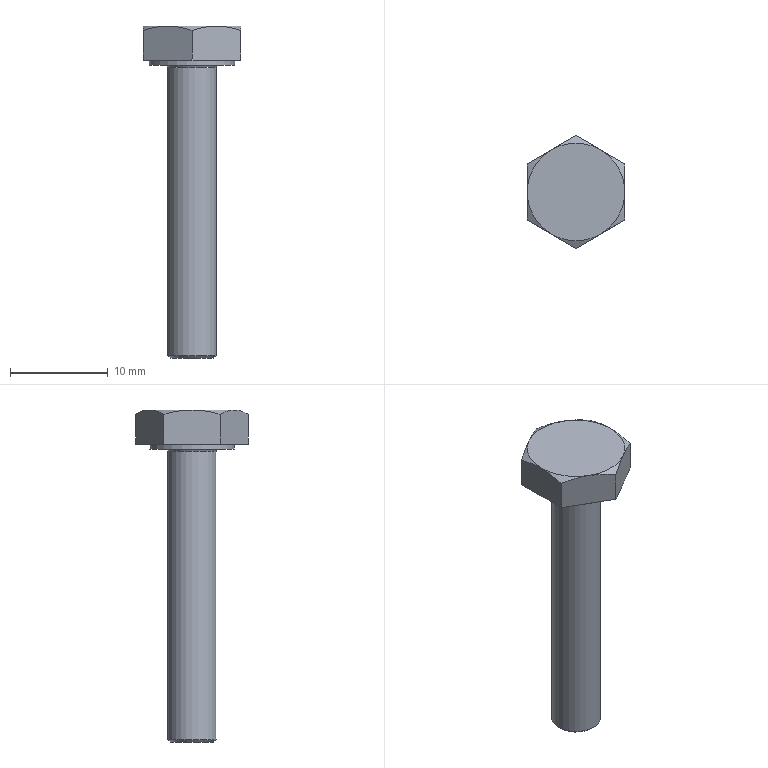Component | NX | BOLT_M6X30 | 1 solid | 20 faces | volume 921 mm3 | plane 10 | cone 7 | cylinder 2 | torus 1 | commonest cylinder face diameters 8.74 x1 5 x1